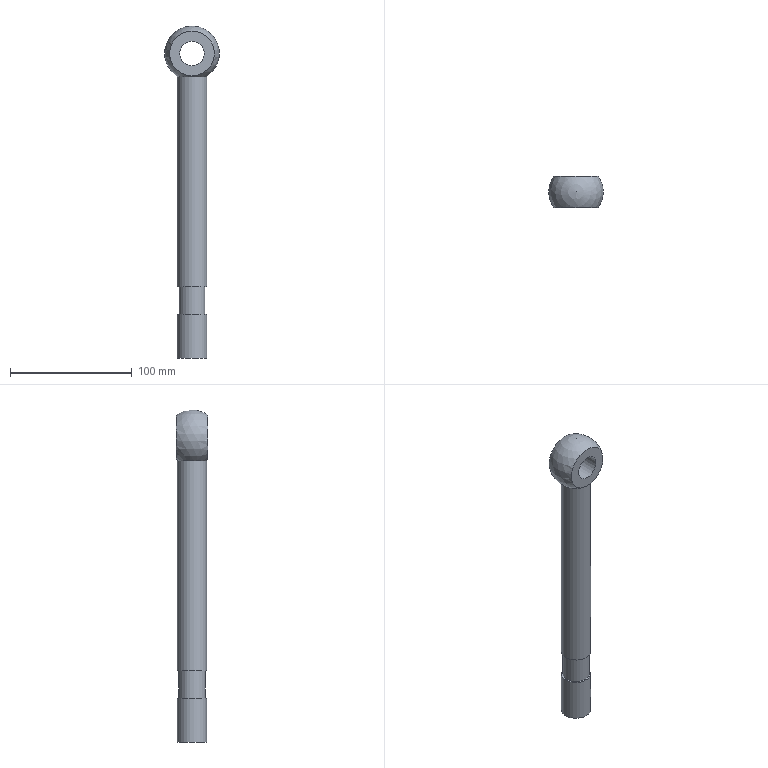Component | NX | HINGE_SCREW | 1 solid | 10 faces | box 45 x 26 x 272.5 mm | volume 130299 mm3 | plane 5 | cylinder 4 | sphere 1 | commonest cylinder face diameters 24 x2 20 x1 21.564 x1
STEP:
#1=CARTESIAN_POINT('',(0.,0.,0.));
#2=DIRECTION('',(0.,0.,1.));
#3=DIRECTION('',(1.,0.,0.));
#4=AXIS2_PLACEMENT_3D('',#1,#2,#3);
#5=CARTESIAN_POINT('',(-170.,-92.,248.467));
#6=VERTEX_POINT('',#5);
#7=CARTESIAN_POINT('',(-170.,-80.,248.467));
#8=DIRECTION('',(0.,0.,-1.));
#9=DIRECTION('',(0.,-1.,0.));
#10=AXIS2_PLACEMENT_3D('',#7,#8,#9);
#11=CIRCLE('',#10,12.);
#12=CARTESIAN_POINT('',(-170.,-80.,267.5));
#13=DIRECTION('',(0.,0.,1.));
#14=DIRECTION('',(0.,-1.,0.));
#15=AXIS2_PLACEMENT_3D('',#12,#13,#14);
#16=SPHERICAL_SURFACE('',#15,22.5);
#17=CARTESIAN_POINT('',(6.283,-1.008));
#18=CARTESIAN_POINT('',(6.188,-1.008));
#19=CARTESIAN_POINT('',(5.998,-1.008));
#20=CARTESIAN_POINT('',(5.712,-1.008));
#21=CARTESIAN_POINT('',(5.426,-1.008));
#22=CARTESIAN_POINT('',(5.141,-1.008));
#23=CARTESIAN_POINT('',(4.855,-1.008));
#24=CARTESIAN_POINT('',(4.57,-1.008));
#25=CARTESIAN_POINT('',(4.284,-1.008));
#26=CARTESIAN_POINT('',(3.998,-1.008));
#27=CARTESIAN_POINT('',(3.713,-1.008));
#28=CARTESIAN_POINT('',(3.427,-1.008));
#29=CARTESIAN_POINT('',(3.142,-1.008));
#30=CARTESIAN_POINT('',(2.856,-1.008));
#31=CARTESIAN_POINT('',(2.57,-1.008));
#32=CARTESIAN_POINT('',(2.285,-1.008));
#33=CARTESIAN_POINT('',(1.999,-1.008));
#34=CARTESIAN_POINT('',(1.714,-1.008));
#35=CARTESIAN_POINT('',(1.428,-1.008));
#36=CARTESIAN_POINT('',(1.142,-1.008));
#37=CARTESIAN_POINT('',(0.8568,-1.008));
#38=CARTESIAN_POINT('',(0.5712,-1.008));
#39=CARTESIAN_POINT('',(0.2856,-1.008));
#40=CARTESIAN_POINT('',(0.0952,-1.008));
#41=CARTESIAN_POINT('',(0.,-1.008));
#42=B_SPLINE_CURVE_WITH_KNOTS('',3,(#17,#18,#19,#20,#21,#22,#23,#24,#25,#26,#27,#28,#29,#30,#31,#32,#33,#34,#35,#36,#37,#38,#39,#40,#41),.UNSPECIFIED.,.F.,.F.,(4,1,1,1,1,1,1,1,1,1,1,1,1,1,1,1,1,1,1,1,1,1,4),(0.,0.2856,0.5712,0.8568,1.142,1.428,1.714,1.999,2.285,2.57,2.856,3.142,3.427,3.713,3.998,4.284,4.57,4.855,5.141,5.426,5.712,5.998,6.283),.QUASI_UNIFORM_KNOTS.);
#43=(GEOMETRIC_REPRESENTATION_CONTEXT(2)PARAMETRIC_REPRESENTATION_CONTEXT()REPRESENTATION_CONTEXT('',''));
#44=DEFINITIONAL_REPRESENTATION('',(#42),#43);
#45=PCURVE('',#16,#44);
#46=CARTESIAN_POINT('',(-170.,-80.,17.5));
#47=DIRECTION('',(0.,0.,1.));
#48=DIRECTION('',(0.,-1.,0.));
#49=AXIS2_PLACEMENT_3D('',#46,#47,#48);
#50=CYLINDRICAL_SURFACE('',#49,12.);
#51=CARTESIAN_POINT('',(6.283,230.967));
#52=DIRECTION('',(-1.,0.));
#53=VECTOR('',#52,1.);
#54=LINE('',#51,#53);
#55=(GEOMETRIC_REPRESENTATION_CONTEXT(2)PARAMETRIC_REPRESENTATION_CONTEXT()REPRESENTATION_CONTEXT('',''));
#56=DEFINITIONAL_REPRESENTATION('',(#54),#55);
#57=PCURVE('',#50,#56);
#58=SURFACE_CURVE('',#11,(#45,#57),.PCURVE_S1.);
#59=EDGE_CURVE('',#6,#6,#58,.T.);
#60=ORIENTED_EDGE('',*,*,#59,.F.);
#61=CARTESIAN_POINT('',(-170.,-93.,249.136));
#62=VERTEX_POINT('',#61);
#63=CARTESIAN_POINT('',(-170.,-92.,248.467));
#64=CARTESIAN_POINT('',(-170.,-92.339,248.681));
#65=CARTESIAN_POINT('',(-170.,-92.673,248.904));
#66=CARTESIAN_POINT('',(-170.,-93.,249.136));
#67=B_SPLINE_CURVE_WITH_KNOTS('',3,(#63,#64,#65,#66),.UNSPECIFIED.,.F.,.F.,(4,4),(-1.008,-0.9548),.PIECEWISE_BEZIER_KNOTS.);
#68=CARTESIAN_POINT('',(6.283,0.));
#69=DIRECTION('',(0.,1.));
#70=VECTOR('',#69,1.);
#71=LINE('',#68,#70);
#72=(GEOMETRIC_REPRESENTATION_CONTEXT(2)PARAMETRIC_REPRESENTATION_CONTEXT()REPRESENTATION_CONTEXT('',''));
#73=DEFINITIONAL_REPRESENTATION('',(#71),#72);
#74=PCURVE('',#16,#73);
#75=CARTESIAN_POINT('',(0.,0.));
#76=DIRECTION('',(0.,1.));
#77=VECTOR('',#76,1.);
#78=LINE('',#75,#77);
#79=(GEOMETRIC_REPRESENTATION_CONTEXT(2)PARAMETRIC_REPRESENTATION_CONTEXT()REPRESENTATION_CONTEXT('',''));
#80=DEFINITIONAL_REPRESENTATION('',(#78),#79);
#81=PCURVE('',#16,#80);
#82=SEAM_CURVE('',#67,(#74,#81),.PCURVE_S1.);
#83=EDGE_CURVE('',#6,#62,#82,.T.);
#84=ORIENTED_EDGE('',*,*,#83,.T.);
#85=CARTESIAN_POINT('',(-170.,-93.,285.864));
#86=VERTEX_POINT('',#85);
#87=CARTESIAN_POINT('',(-170.,-93.,267.5));
#88=DIRECTION('',(0.,1.,0.));
#89=DIRECTION('',(0.,0.,-1.));
#90=AXIS2_PLACEMENT_3D('',#87,#88,#89);
#91=CIRCLE('',#90,18.364);
#92=CARTESIAN_POINT('',(6.283,-0.9548));
#93=CARTESIAN_POINT('',(6.14,-0.9552));
#94=CARTESIAN_POINT('',(5.887,-0.9144));
#95=CARTESIAN_POINT('',(5.611,-0.7647));
#96=CARTESIAN_POINT('',(5.453,-0.5678));
#97=CARTESIAN_POINT('',(5.365,-0.3477));
#98=CARTESIAN_POINT('',(5.327,-0.1169));
#99=CARTESIAN_POINT('',(5.327,0.1169));
#100=CARTESIAN_POINT('',(5.366,0.3477));
#101=CARTESIAN_POINT('',(5.453,0.5678));
#102=CARTESIAN_POINT('',(5.612,0.7647));
#103=CARTESIAN_POINT('',(5.883,0.9147));
#104=CARTESIAN_POINT('',(6.283,0.9749));
#105=CARTESIAN_POINT('',(6.684,0.9147));
#106=CARTESIAN_POINT('',(6.954,0.7647));
#107=CARTESIAN_POINT('',(7.113,0.5678));
#108=CARTESIAN_POINT('',(7.201,0.3477));
#109=CARTESIAN_POINT('',(7.24,0.1169));
#110=CARTESIAN_POINT('',(7.24,-0.1169));
#111=CARTESIAN_POINT('',(7.201,-0.3477));
#112=CARTESIAN_POINT('',(7.113,-0.5678));
#113=CARTESIAN_POINT('',(6.955,-0.7647));
#114=CARTESIAN_POINT('',(6.679,-0.9144));
#115=CARTESIAN_POINT('',(6.427,-0.9552));
#116=CARTESIAN_POINT('',(6.283,-0.9548));
#117=B_SPLINE_CURVE_WITH_KNOTS('',3,(#92,#93,#94,#95,#96,#97,#98,#99,#100,#101,#102,#103,#104,#105,#106,#107,#108,#109,#110,#111,#112,#113,#114,#115,#116),.UNSPECIFIED.,.T.,.F.,(4,1,1,1,1,1,1,1,1,1,1,1,1,1,1,1,1,1,1,1,1,1,4),(0.,0.2856,0.5712,0.8568,1.142,1.428,1.714,1.999,2.285,2.57,2.856,3.142,3.427,3.713,3.998,4.284,4.57,4.855,5.141,5.426,5.712,5.998,6.283),.QUASI_UNIFORM_KNOTS.);
#118=(GEOMETRIC_REPRESENTATION_CONTEXT(2)PARAMETRIC_REPRESENTATION_CONTEXT()REPRESENTATION_CONTEXT('',''));
#119=DEFINITIONAL_REPRESENTATION('',(#117),#118);
#120=PCURVE('',#16,#119);
#121=CARTESIAN_POINT('',(-170.,-93.,267.5));
#122=DIRECTION('',(0.,-1.,0.));
#123=DIRECTION('',(0.,0.,-1.));
#124=AXIS2_PLACEMENT_3D('',#121,#122,#123);
#125=PLANE('',#124);
#126=CARTESIAN_POINT('',(18.364,0.));
#127=CARTESIAN_POINT('',(18.364,-31.808));
#128=CARTESIAN_POINT('',(-9.182,-15.904));
#129=CARTESIAN_POINT('',(-36.729,-0.));
#130=CARTESIAN_POINT('',(-9.182,15.904));
#131=CARTESIAN_POINT('',(18.364,31.808));
#132=CARTESIAN_POINT('',(18.364,0.));
#133=(BOUNDED_CURVE()B_SPLINE_CURVE(2,(#126,#127,#128,#129,#130,#131,#132),.UNSPECIFIED.,.T.,.F.)B_SPLINE_CURVE_WITH_KNOTS((1,2,2,2,2,1),(-2.094,0.,2.094,4.189,6.283,8.378),.UNSPECIFIED.)CURVE()GEOMETRIC_REPRESENTATION_ITEM()RATIONAL_B_SPLINE_CURVE((1.,0.5,1.,0.5,1.,0.5,1.))REPRESENTATION_ITEM(''));
#134=(GEOMETRIC_REPRESENTATION_CONTEXT(2)PARAMETRIC_REPRESENTATION_CONTEXT()REPRESENTATION_CONTEXT('',''));
#135=DEFINITIONAL_REPRESENTATION('',(#133),#134);
#136=PCURVE('',#125,#135);
#137=SURFACE_CURVE('',#91,(#120,#136),.PCURVE_S1.);
#138=EDGE_CURVE('',#62,#86,#137,.T.);
#139=ORIENTED_EDGE('',*,*,#138,.T.);
#140=CARTESIAN_POINT('',(-170.,-80.,290.));
#141=VERTEX_POINT('',#140);
#142=CARTESIAN_POINT('',(-170.,-93.,285.864));
#143=CARTESIAN_POINT('',(-170.,-90.737,287.466));
#144=CARTESIAN_POINT('',(-170.,-88.228,288.719));
#145=CARTESIAN_POINT('',(-170.,-85.544,289.573));
#146=CARTESIAN_POINT('',(-170.,-82.772,290.));
#147=CARTESIAN_POINT('',(-170.,-80.,290.));
#148=B_SPLINE_CURVE_WITH_KNOTS('',5,(#142,#143,#144,#145,#146,#147),.UNSPECIFIED.,.F.,.F.,(6,6),(0.9548,1.571),.PIECEWISE_BEZIER_KNOTS.);
#149=CARTESIAN_POINT('',(6.283,0.));
#150=DIRECTION('',(0.,1.));
#151=VECTOR('',#150,1.);
#152=LINE('',#149,#151);
#153=(GEOMETRIC_REPRESENTATION_CONTEXT(2)PARAMETRIC_REPRESENTATION_CONTEXT()REPRESENTATION_CONTEXT('',''));
#154=DEFINITIONAL_REPRESENTATION('',(#152),#153);
#155=PCURVE('',#16,#154);
#156=CARTESIAN_POINT('',(0.,0.));
#157=DIRECTION('',(0.,1.));
#158=VECTOR('',#157,1.);
#159=LINE('',#156,#158);
#160=(GEOMETRIC_REPRESENTATION_CONTEXT(2)PARAMETRIC_REPRESENTATION_CONTEXT()REPRESENTATION_CONTEXT('',''));
#161=DEFINITIONAL_REPRESENTATION('',(#159),#160);
#162=PCURVE('',#16,#161);
#163=SEAM_CURVE('',#148,(#155,#162),.PCURVE_S1.);
#164=EDGE_CURVE('',#86,#141,#163,.T.);
#165=ORIENTED_EDGE('',*,*,#164,.T.);
#166=ORIENTED_EDGE('',*,*,#164,.F.);
#167=CARTESIAN_POINT('',(-170.,-93.,267.5));
#168=DIRECTION('',(0.,1.,0.));
#169=DIRECTION('',(0.,0.,-1.));
#170=AXIS2_PLACEMENT_3D('',#167,#168,#169);
#171=CIRCLE('',#170,18.364);
#172=CARTESIAN_POINT('',(0.,-0.9548));
#173=CARTESIAN_POINT('',(-0.1436,-0.9552));
#174=CARTESIAN_POINT('',(-0.3958,-0.9144));
#175=CARTESIAN_POINT('',(-0.672,-0.7647));
#176=CARTESIAN_POINT('',(-0.8297,-0.5678));
#177=CARTESIAN_POINT('',(-0.9177,-0.3477));
#178=CARTESIAN_POINT('',(-0.9564,-0.1169));
#179=CARTESIAN_POINT('',(-0.9564,0.1169));
#180=CARTESIAN_POINT('',(-0.9176,0.3477));
#181=CARTESIAN_POINT('',(-0.83,0.5678));
#182=CARTESIAN_POINT('',(-0.6707,0.7647));
#183=CARTESIAN_POINT('',(-0.4005,0.9147));
#184=CARTESIAN_POINT('',(-0.,0.9749));
#185=CARTESIAN_POINT('',(0.4005,0.9147));
#186=CARTESIAN_POINT('',(0.6707,0.7647));
#187=CARTESIAN_POINT('',(0.83,0.5678));
#188=CARTESIAN_POINT('',(0.9176,0.3477));
#189=CARTESIAN_POINT('',(0.9564,0.1169));
#190=CARTESIAN_POINT('',(0.9564,-0.1169));
#191=CARTESIAN_POINT('',(0.9177,-0.3477));
#192=CARTESIAN_POINT('',(0.8297,-0.5678));
#193=CARTESIAN_POINT('',(0.672,-0.7647));
#194=CARTESIAN_POINT('',(0.3958,-0.9144));
#195=CARTESIAN_POINT('',(0.1436,-0.9552));
#196=CARTESIAN_POINT('',(0.,-0.9548));
#197=B_SPLINE_CURVE_WITH_KNOTS('',3,(#172,#173,#174,#175,#176,#177,#178,#179,#180,#181,#182,#183,#184,#185,#186,#187,#188,#189,#190,#191,#192,#193,#194,#195,#196),.UNSPECIFIED.,.T.,.F.,(4,1,1,1,1,1,1,1,1,1,1,1,1,1,1,1,1,1,1,1,1,1,4),(0.,0.2856,0.5712,0.8568,1.142,1.428,1.714,1.999,2.285,2.57,2.856,3.142,3.427,3.713,3.998,4.284,4.57,4.855,5.141,5.426,5.712,5.998,6.283),.QUASI_UNIFORM_KNOTS.);
#198=(GEOMETRIC_REPRESENTATION_CONTEXT(2)PARAMETRIC_REPRESENTATION_CONTEXT()REPRESENTATION_CONTEXT('',''));
#199=DEFINITIONAL_REPRESENTATION('',(#197),#198);
#200=PCURVE('',#16,#199);
#201=CARTESIAN_POINT('',(18.364,0.));
#202=CARTESIAN_POINT('',(18.364,-31.808));
#203=CARTESIAN_POINT('',(-9.182,-15.904));
#204=CARTESIAN_POINT('',(-36.729,-0.));
#205=CARTESIAN_POINT('',(-9.182,15.904));
#206=CARTESIAN_POINT('',(18.364,31.808));
#207=CARTESIAN_POINT('',(18.364,0.));
#208=(BOUNDED_CURVE()B_SPLINE_CURVE(2,(#201,#202,#203,#204,#205,#206,#207),.UNSPECIFIED.,.T.,.F.)B_SPLINE_CURVE_WITH_KNOTS((1,2,2,2,2,1),(-2.094,0.,2.094,4.189,6.283,8.378),.UNSPECIFIED.)CURVE()GEOMETRIC_REPRESENTATION_ITEM()RATIONAL_B_SPLINE_CURVE((1.,0.5,1.,0.5,1.,0.5,1.))REPRESENTATION_ITEM(''));
#209=(GEOMETRIC_REPRESENTATION_CONTEXT(2)PARAMETRIC_REPRESENTATION_CONTEXT()REPRESENTATION_CONTEXT('',''));
#210=DEFINITIONAL_REPRESENTATION('',(#208),#209);
#211=PCURVE('',#125,#210);
#212=SURFACE_CURVE('',#171,(#200,#211),.PCURVE_S1.);
#213=EDGE_CURVE('',#86,#62,#212,.T.);
#214=ORIENTED_EDGE('',*,*,#213,.T.);
#215=ORIENTED_EDGE('',*,*,#83,.F.);
#216=EDGE_LOOP('',(#60,#84,#139,#165,#166,#214,#215));
#217=FACE_BOUND('',#216,.T.);
#218=CARTESIAN_POINT('',(-170.,-67.,285.864));
#219=VERTEX_POINT('',#218);
#220=CARTESIAN_POINT('',(-170.,-67.,267.5));
#221=DIRECTION('',(0.,-1.,0.));
#222=DIRECTION('',(0.,0.,1.));
#223=AXIS2_PLACEMENT_3D('',#220,#221,#222);
#224=CIRCLE('',#223,18.364);
#225=CARTESIAN_POINT('',(3.142,0.9548));
#226=CARTESIAN_POINT('',(3.285,0.9552));
#227=CARTESIAN_POINT('',(3.537,0.9144));
#228=CARTESIAN_POINT('',(3.814,0.7647));
#229=CARTESIAN_POINT('',(3.971,0.5678));
#230=CARTESIAN_POINT('',(4.059,0.3477));
#231=CARTESIAN_POINT('',(4.098,0.1169));
#232=CARTESIAN_POINT('',(4.098,-0.1169));
#233=CARTESIAN_POINT('',(4.059,-0.3477));
#234=CARTESIAN_POINT('',(3.972,-0.5678));
#235=CARTESIAN_POINT('',(3.812,-0.7647));
#236=CARTESIAN_POINT('',(3.542,-0.9147));
#237=CARTESIAN_POINT('',(3.142,-0.9749));
#238=CARTESIAN_POINT('',(2.741,-0.9147));
#239=CARTESIAN_POINT('',(2.471,-0.7647));
#240=CARTESIAN_POINT('',(2.312,-0.5678));
#241=CARTESIAN_POINT('',(2.224,-0.3477));
#242=CARTESIAN_POINT('',(2.185,-0.1169));
#243=CARTESIAN_POINT('',(2.185,0.1169));
#244=CARTESIAN_POINT('',(2.224,0.3477));
#245=CARTESIAN_POINT('',(2.312,0.5678));
#246=CARTESIAN_POINT('',(2.47,0.7647));
#247=CARTESIAN_POINT('',(2.746,0.9144));
#248=CARTESIAN_POINT('',(2.998,0.9552));
#249=CARTESIAN_POINT('',(3.142,0.9548));
#250=B_SPLINE_CURVE_WITH_KNOTS('',3,(#225,#226,#227,#228,#229,#230,#231,#232,#233,#234,#235,#236,#237,#238,#239,#240,#241,#242,#243,#244,#245,#246,#247,#248,#249),.UNSPECIFIED.,.T.,.F.,(4,1,1,1,1,1,1,1,1,1,1,1,1,1,1,1,1,1,1,1,1,1,4),(0.,0.2856,0.5712,0.8568,1.142,1.428,1.714,1.999,2.285,2.57,2.856,3.142,3.427,3.713,3.998,4.284,4.57,4.855,5.141,5.426,5.712,5.998,6.283),.QUASI_UNIFORM_KNOTS.);
#251=(GEOMETRIC_REPRESENTATION_CONTEXT(2)PARAMETRIC_REPRESENTATION_CONTEXT()REPRESENTATION_CONTEXT('',''));
#252=DEFINITIONAL_REPRESENTATION('',(#250),#251);
#253=PCURVE('',#16,#252);
#254=CARTESIAN_POINT('',(-170.,-67.,267.5));
#255=DIRECTION('',(0.,1.,0.));
#256=DIRECTION('',(0.,0.,1.));
#257=AXIS2_PLACEMENT_3D('',#254,#255,#256);
#258=PLANE('',#257);
#259=CARTESIAN_POINT('',(18.364,0.));
#260=CARTESIAN_POINT('',(18.364,-31.808));
#261=CARTESIAN_POINT('',(-9.182,-15.904));
#262=CARTESIAN_POINT('',(-36.729,-0.));
#263=CARTESIAN_POINT('',(-9.182,15.904));
#264=CARTESIAN_POINT('',(18.364,31.808));
#265=CARTESIAN_POINT('',(18.364,0.));
#266=(BOUNDED_CURVE()B_SPLINE_CURVE(2,(#259,#260,#261,#262,#263,#264,#265),.UNSPECIFIED.,.T.,.F.)B_SPLINE_CURVE_WITH_KNOTS((1,2,2,2,2,1),(-2.094,0.,2.094,4.189,6.283,8.378),.UNSPECIFIED.)CURVE()GEOMETRIC_REPRESENTATION_ITEM()RATIONAL_B_SPLINE_CURVE((1.,0.5,1.,0.5,1.,0.5,1.))REPRESENTATION_ITEM(''));
#267=(GEOMETRIC_REPRESENTATION_CONTEXT(2)PARAMETRIC_REPRESENTATION_CONTEXT()REPRESENTATION_CONTEXT('',''));
#268=DEFINITIONAL_REPRESENTATION('',(#266),#267);
#269=PCURVE('',#258,#268);
#270=SURFACE_CURVE('',#224,(#253,#269),.PCURVE_S1.);
#271=EDGE_CURVE('',#219,#219,#270,.T.);
#272=ORIENTED_EDGE('',*,*,#271,.T.);
#273=EDGE_LOOP('',(#272));
#274=FACE_BOUND('',#273,.T.);
#275=ADVANCED_FACE('',(#217,#274),#16,.T.);
#276=CARTESIAN_POINT('',(-170.,-93.,277.5));
#277=VERTEX_POINT('',#276);
#278=CARTESIAN_POINT('',(-170.,-93.,267.5));
#279=DIRECTION('',(0.,1.,0.));
#280=DIRECTION('',(0.,0.,1.));
#281=AXIS2_PLACEMENT_3D('',#278,#279,#280);
#282=CIRCLE('',#281,10.);
#283=CARTESIAN_POINT('',(-10.,0.));
#284=CARTESIAN_POINT('',(-10.,17.321));
#285=CARTESIAN_POINT('',(5.,8.66));
#286=CARTESIAN_POINT('',(20.,0.));
#287=CARTESIAN_POINT('',(5.,-8.66));
#288=CARTESIAN_POINT('',(-10.,-17.321));
#289=CARTESIAN_POINT('',(-10.,0.));
#290=(BOUNDED_CURVE()B_SPLINE_CURVE(2,(#283,#284,#285,#286,#287,#288,#289),.UNSPECIFIED.,.T.,.F.)B_SPLINE_CURVE_WITH_KNOTS((1,2,2,2,2,1),(-2.094,0.,2.094,4.189,6.283,8.378),.UNSPECIFIED.)CURVE()GEOMETRIC_REPRESENTATION_ITEM()RATIONAL_B_SPLINE_CURVE((1.,0.5,1.,0.5,1.,0.5,1.))REPRESENTATION_ITEM(''));
#291=(GEOMETRIC_REPRESENTATION_CONTEXT(2)PARAMETRIC_REPRESENTATION_CONTEXT()REPRESENTATION_CONTEXT('',''));
#292=DEFINITIONAL_REPRESENTATION('',(#290),#291);
#293=PCURVE('',#125,#292);
#294=CARTESIAN_POINT('',(-170.,-93.,267.5));
#295=DIRECTION('',(0.,1.,0.));
#296=DIRECTION('',(0.,0.,1.));
#297=AXIS2_PLACEMENT_3D('',#294,#295,#296);
#298=CYLINDRICAL_SURFACE('',#297,10.);
#299=CARTESIAN_POINT('',(0.,0.));
#300=DIRECTION('',(1.,0.));
#301=VECTOR('',#300,1.);
#302=LINE('',#299,#301);
#303=(GEOMETRIC_REPRESENTATION_CONTEXT(2)PARAMETRIC_REPRESENTATION_CONTEXT()REPRESENTATION_CONTEXT('',''));
#304=DEFINITIONAL_REPRESENTATION('',(#302),#303);
#305=PCURVE('',#298,#304);
#306=SURFACE_CURVE('',#282,(#293,#305),.PCURVE_S1.);
#307=EDGE_CURVE('',#277,#277,#306,.T.);
#308=ORIENTED_EDGE('',*,*,#307,.T.);
#309=EDGE_LOOP('',(#308));
#310=FACE_BOUND('',#309,.T.);
#311=ORIENTED_EDGE('',*,*,#138,.F.);
#312=ORIENTED_EDGE('',*,*,#213,.F.);
#313=EDGE_LOOP('',(#311,#312));
#314=FACE_BOUND('',#313,.T.);
#315=ADVANCED_FACE('',(#310,#314),#125,.T.);
#316=CARTESIAN_POINT('',(-170.,-67.,277.5));
#317=VERTEX_POINT('',#316);
#318=CARTESIAN_POINT('',(-170.,-67.,267.5));
#319=DIRECTION('',(0.,1.,0.));
#320=DIRECTION('',(0.,0.,1.));
#321=AXIS2_PLACEMENT_3D('',#318,#319,#320);
#322=CIRCLE('',#321,10.);
#323=CARTESIAN_POINT('',(0.,0.));
#324=DIRECTION('',(1.,0.));
#325=AXIS2_PLACEMENT_2D('',#323,#324);
#326=CIRCLE('',#325,10.);
#327=(GEOMETRIC_REPRESENTATION_CONTEXT(2)PARAMETRIC_REPRESENTATION_CONTEXT()REPRESENTATION_CONTEXT('',''));
#328=DEFINITIONAL_REPRESENTATION('',(#326),#327);
#329=PCURVE('',#258,#328);
#330=CARTESIAN_POINT('',(0.,26.));
#331=DIRECTION('',(1.,0.));
#332=VECTOR('',#331,1.);
#333=LINE('',#330,#332);
#334=(GEOMETRIC_REPRESENTATION_CONTEXT(2)PARAMETRIC_REPRESENTATION_CONTEXT()REPRESENTATION_CONTEXT('',''));
#335=DEFINITIONAL_REPRESENTATION('',(#333),#334);
#336=PCURVE('',#298,#335);
#337=SURFACE_CURVE('',#322,(#329,#336),.PCURVE_S1.);
#338=EDGE_CURVE('',#317,#317,#337,.T.);
#339=ORIENTED_EDGE('',*,*,#338,.F.);
#340=EDGE_LOOP('',(#339));
#341=FACE_BOUND('',#340,.T.);
#342=ORIENTED_EDGE('',*,*,#271,.F.);
#343=EDGE_LOOP('',(#342));
#344=FACE_BOUND('',#343,.T.);
#345=ADVANCED_FACE('',(#341,#344),#258,.T.);
#346=CARTESIAN_POINT('',(-170.,-92.,76.));
#347=VERTEX_POINT('',#346);
#348=CARTESIAN_POINT('',(-170.,-80.,76.));
#349=DIRECTION('',(0.,0.,-1.));
#350=DIRECTION('',(0.,-1.,0.));
#351=AXIS2_PLACEMENT_3D('',#348,#349,#350);
#352=CIRCLE('',#351,12.);
#353=CARTESIAN_POINT('',(6.283,58.5));
#354=DIRECTION('',(-1.,0.));
#355=VECTOR('',#354,1.);
#356=LINE('',#353,#355);
#357=(GEOMETRIC_REPRESENTATION_CONTEXT(2)PARAMETRIC_REPRESENTATION_CONTEXT()REPRESENTATION_CONTEXT('',''));
#358=DEFINITIONAL_REPRESENTATION('',(#356),#357);
#359=PCURVE('',#50,#358);
#360=CARTESIAN_POINT('',(-170.,-80.,76.));
#361=DIRECTION('',(0.,0.,1.));
#362=DIRECTION('',(0.,-1.,0.));
#363=AXIS2_PLACEMENT_3D('',#360,#361,#362);
#364=PLANE('',#363);
#365=CARTESIAN_POINT('',(12.,0.));
#366=CARTESIAN_POINT('',(12.,-20.785));
#367=CARTESIAN_POINT('',(-6.,-10.392));
#368=CARTESIAN_POINT('',(-24.,-0.));
#369=CARTESIAN_POINT('',(-6.,10.392));
#370=CARTESIAN_POINT('',(12.,20.785));
#371=CARTESIAN_POINT('',(12.,0.));
#372=(BOUNDED_CURVE()B_SPLINE_CURVE(2,(#365,#366,#367,#368,#369,#370,#371),.UNSPECIFIED.,.T.,.F.)B_SPLINE_CURVE_WITH_KNOTS((1,2,2,2,2,1),(-2.094,0.,2.094,4.189,6.283,8.378),.UNSPECIFIED.)CURVE()GEOMETRIC_REPRESENTATION_ITEM()RATIONAL_B_SPLINE_CURVE((1.,0.5,1.,0.5,1.,0.5,1.))REPRESENTATION_ITEM(''));
#373=(GEOMETRIC_REPRESENTATION_CONTEXT(2)PARAMETRIC_REPRESENTATION_CONTEXT()REPRESENTATION_CONTEXT('',''));
#374=DEFINITIONAL_REPRESENTATION('',(#372),#373);
#375=PCURVE('',#364,#374);
#376=SURFACE_CURVE('',#352,(#359,#375),.PCURVE_S1.);
#377=EDGE_CURVE('',#347,#347,#376,.T.);
#378=ORIENTED_EDGE('',*,*,#377,.F.);
#379=CARTESIAN_POINT('',(-170.,-92.,76.));
#380=CARTESIAN_POINT('',(-170.,-92.,248.467));
#381=B_SPLINE_CURVE_WITH_KNOTS('',1,(#379,#380),.UNSPECIFIED.,.F.,.F.,(2,2),(58.5,230.967),.PIECEWISE_BEZIER_KNOTS.);
#382=CARTESIAN_POINT('',(6.283,0.));
#383=DIRECTION('',(0.,1.));
#384=VECTOR('',#383,1.);
#385=LINE('',#382,#384);
#386=(GEOMETRIC_REPRESENTATION_CONTEXT(2)PARAMETRIC_REPRESENTATION_CONTEXT()REPRESENTATION_CONTEXT('',''));
#387=DEFINITIONAL_REPRESENTATION('',(#385),#386);
#388=PCURVE('',#50,#387);
#389=CARTESIAN_POINT('',(0.,0.));
#390=DIRECTION('',(0.,1.));
#391=VECTOR('',#390,1.);
#392=LINE('',#389,#391);
#393=(GEOMETRIC_REPRESENTATION_CONTEXT(2)PARAMETRIC_REPRESENTATION_CONTEXT()REPRESENTATION_CONTEXT('',''));
#394=DEFINITIONAL_REPRESENTATION('',(#392),#393);
#395=PCURVE('',#50,#394);
#396=SEAM_CURVE('',#381,(#388,#395),.PCURVE_S1.);
#397=EDGE_CURVE('',#347,#6,#396,.T.);
#398=ORIENTED_EDGE('',*,*,#397,.T.);
#399=ORIENTED_EDGE('',*,*,#59,.T.);
#400=ORIENTED_EDGE('',*,*,#397,.F.);
#401=EDGE_LOOP('',(#378,#398,#399,#400));
#402=FACE_BOUND('',#401,.T.);
#403=ADVANCED_FACE('',(#402),#50,.T.);
#404=ORIENTED_EDGE('',*,*,#338,.F.);
#405=CARTESIAN_POINT('',(-170.,-93.,277.5));
#406=CARTESIAN_POINT('',(-170.,-67.,277.5));
#407=B_SPLINE_CURVE_WITH_KNOTS('',1,(#405,#406),.UNSPECIFIED.,.F.,.F.,(2,2),(0.,26.),.PIECEWISE_BEZIER_KNOTS.);
#408=CARTESIAN_POINT('',(0.,0.));
#409=DIRECTION('',(0.,1.));
#410=VECTOR('',#409,1.);
#411=LINE('',#408,#410);
#412=(GEOMETRIC_REPRESENTATION_CONTEXT(2)PARAMETRIC_REPRESENTATION_CONTEXT()REPRESENTATION_CONTEXT('',''));
#413=DEFINITIONAL_REPRESENTATION('',(#411),#412);
#414=PCURVE('',#298,#413);
#415=CARTESIAN_POINT('',(6.283,0.));
#416=DIRECTION('',(0.,1.));
#417=VECTOR('',#416,1.);
#418=LINE('',#415,#417);
#419=(GEOMETRIC_REPRESENTATION_CONTEXT(2)PARAMETRIC_REPRESENTATION_CONTEXT()REPRESENTATION_CONTEXT('',''));
#420=DEFINITIONAL_REPRESENTATION('',(#418),#419);
#421=PCURVE('',#298,#420);
#422=SEAM_CURVE('',#407,(#414,#421),.PCURVE_S1.);
#423=EDGE_CURVE('',#277,#317,#422,.T.);
#424=ORIENTED_EDGE('',*,*,#423,.F.);
#425=ORIENTED_EDGE('',*,*,#307,.T.);
#426=ORIENTED_EDGE('',*,*,#423,.T.);
#427=EDGE_LOOP('',(#404,#424,#425,#426));
#428=FACE_BOUND('',#427,.F.);
#429=ADVANCED_FACE('',(#428),#298,.F.);
#430=CARTESIAN_POINT('',(-170.,-90.782,76.));
#431=VERTEX_POINT('',#430);
#432=CARTESIAN_POINT('',(-170.,-80.,76.));
#433=DIRECTION('',(0.,0.,1.));
#434=DIRECTION('',(0.,-1.,0.));
#435=AXIS2_PLACEMENT_3D('',#432,#433,#434);
#436=CIRCLE('',#435,10.782);
#437=CARTESIAN_POINT('',(-170.,-80.,76.));
#438=DIRECTION('',(0.,0.,-1.));
#439=DIRECTION('',(0.,1.,0.));
#440=AXIS2_PLACEMENT_3D('',#437,#438,#439);
#441=CYLINDRICAL_SURFACE('',#440,10.782);
#442=CARTESIAN_POINT('',(9.425,0.));
#443=DIRECTION('',(-1.,0.));
#444=VECTOR('',#443,1.);
#445=LINE('',#442,#444);
#446=(GEOMETRIC_REPRESENTATION_CONTEXT(2)PARAMETRIC_REPRESENTATION_CONTEXT()REPRESENTATION_CONTEXT('',''));
#447=DEFINITIONAL_REPRESENTATION('',(#445),#446);
#448=PCURVE('',#441,#447);
#449=CARTESIAN_POINT('',(0.,0.));
#450=DIRECTION('',(1.,0.));
#451=AXIS2_PLACEMENT_2D('',#449,#450);
#452=CIRCLE('',#451,10.782);
#453=(GEOMETRIC_REPRESENTATION_CONTEXT(2)PARAMETRIC_REPRESENTATION_CONTEXT()REPRESENTATION_CONTEXT('',''));
#454=DEFINITIONAL_REPRESENTATION('',(#452),#453);
#455=PCURVE('',#364,#454);
#456=SURFACE_CURVE('',#436,(#448,#455),.PCURVE_S1.);
#457=EDGE_CURVE('',#431,#431,#456,.T.);
#458=ORIENTED_EDGE('',*,*,#457,.F.);
#459=CARTESIAN_POINT('',(-170.,-90.782,53.5));
#460=VERTEX_POINT('',#459);
#461=CARTESIAN_POINT('',(-170.,-90.782,76.));
#462=CARTESIAN_POINT('',(-170.,-90.782,53.5));
#463=B_SPLINE_CURVE_WITH_KNOTS('',1,(#461,#462),.UNSPECIFIED.,.F.,.F.,(2,2),(0.,22.5),.PIECEWISE_BEZIER_KNOTS.);
#464=CARTESIAN_POINT('',(9.425,0.));
#465=DIRECTION('',(0.,1.));
#466=VECTOR('',#465,1.);
#467=LINE('',#464,#466);
#468=(GEOMETRIC_REPRESENTATION_CONTEXT(2)PARAMETRIC_REPRESENTATION_CONTEXT()REPRESENTATION_CONTEXT('',''));
#469=DEFINITIONAL_REPRESENTATION('',(#467),#468);
#470=PCURVE('',#441,#469);
#471=CARTESIAN_POINT('',(3.142,0.));
#472=DIRECTION('',(0.,1.));
#473=VECTOR('',#472,1.);
#474=LINE('',#471,#473);
#475=(GEOMETRIC_REPRESENTATION_CONTEXT(2)PARAMETRIC_REPRESENTATION_CONTEXT()REPRESENTATION_CONTEXT('',''));
#476=DEFINITIONAL_REPRESENTATION('',(#474),#475);
#477=PCURVE('',#441,#476);
#478=SEAM_CURVE('',#463,(#470,#477),.PCURVE_S1.);
#479=EDGE_CURVE('',#431,#460,#478,.T.);
#480=ORIENTED_EDGE('',*,*,#479,.T.);
#481=CARTESIAN_POINT('',(-170.,-80.,53.5));
#482=DIRECTION('',(0.,0.,1.));
#483=DIRECTION('',(0.,-1.,0.));
#484=AXIS2_PLACEMENT_3D('',#481,#482,#483);
#485=CIRCLE('',#484,10.782);
#486=CARTESIAN_POINT('',(9.425,22.5));
#487=DIRECTION('',(-1.,0.));
#488=VECTOR('',#487,1.);
#489=LINE('',#486,#488);
#490=(GEOMETRIC_REPRESENTATION_CONTEXT(2)PARAMETRIC_REPRESENTATION_CONTEXT()REPRESENTATION_CONTEXT('',''));
#491=DEFINITIONAL_REPRESENTATION('',(#489),#490);
#492=PCURVE('',#441,#491);
#493=CARTESIAN_POINT('',(-170.,-80.,53.5));
#494=DIRECTION('',(0.,0.,1.));
#495=DIRECTION('',(0.,-1.,0.));
#496=AXIS2_PLACEMENT_3D('',#493,#494,#495);
#497=PLANE('',#496);
#498=CARTESIAN_POINT('',(0.,0.));
#499=DIRECTION('',(1.,0.));
#500=AXIS2_PLACEMENT_2D('',#498,#499);
#501=CIRCLE('',#500,10.782);
#502=(GEOMETRIC_REPRESENTATION_CONTEXT(2)PARAMETRIC_REPRESENTATION_CONTEXT()REPRESENTATION_CONTEXT('',''));
#503=DEFINITIONAL_REPRESENTATION('',(#501),#502);
#504=PCURVE('',#497,#503);
#505=SURFACE_CURVE('',#485,(#492,#504),.PCURVE_S1.);
#506=EDGE_CURVE('',#460,#460,#505,.T.);
#507=ORIENTED_EDGE('',*,*,#506,.T.);
#508=ORIENTED_EDGE('',*,*,#479,.F.);
#509=EDGE_LOOP('',(#458,#480,#507,#508));
#510=FACE_BOUND('',#509,.T.);
#511=ADVANCED_FACE('',(#510),#441,.T.);
#512=ORIENTED_EDGE('',*,*,#377,.T.);
#513=EDGE_LOOP('',(#512));
#514=FACE_BOUND('',#513,.T.);
#515=ORIENTED_EDGE('',*,*,#457,.T.);
#516=EDGE_LOOP('',(#515));
#517=FACE_BOUND('',#516,.T.);
#518=ADVANCED_FACE('',(#514,#517),#364,.F.);
#519=CARTESIAN_POINT('',(-170.,-92.,53.5));
#520=VERTEX_POINT('',#519);
#521=CARTESIAN_POINT('',(-170.,-80.,53.5));
#522=DIRECTION('',(0.,0.,-1.));
#523=DIRECTION('',(0.,-1.,0.));
#524=AXIS2_PLACEMENT_3D('',#521,#522,#523);
#525=CIRCLE('',#524,12.);
#526=CARTESIAN_POINT('',(12.,0.));
#527=CARTESIAN_POINT('',(12.,-20.785));
#528=CARTESIAN_POINT('',(-6.,-10.392));
#529=CARTESIAN_POINT('',(-24.,-0.));
#530=CARTESIAN_POINT('',(-6.,10.392));
#531=CARTESIAN_POINT('',(12.,20.785));
#532=CARTESIAN_POINT('',(12.,0.));
#533=(BOUNDED_CURVE()B_SPLINE_CURVE(2,(#526,#527,#528,#529,#530,#531,#532),.UNSPECIFIED.,.T.,.F.)B_SPLINE_CURVE_WITH_KNOTS((1,2,2,2,2,1),(-2.094,0.,2.094,4.189,6.283,8.378),.UNSPECIFIED.)CURVE()GEOMETRIC_REPRESENTATION_ITEM()RATIONAL_B_SPLINE_CURVE((1.,0.5,1.,0.5,1.,0.5,1.))REPRESENTATION_ITEM(''));
#534=(GEOMETRIC_REPRESENTATION_CONTEXT(2)PARAMETRIC_REPRESENTATION_CONTEXT()REPRESENTATION_CONTEXT('',''));
#535=DEFINITIONAL_REPRESENTATION('',(#533),#534);
#536=PCURVE('',#497,#535);
#537=CARTESIAN_POINT('',(-170.,-80.,17.5));
#538=DIRECTION('',(0.,0.,1.));
#539=DIRECTION('',(0.,-1.,0.));
#540=AXIS2_PLACEMENT_3D('',#537,#538,#539);
#541=CYLINDRICAL_SURFACE('',#540,12.);
#542=CARTESIAN_POINT('',(6.283,36.));
#543=DIRECTION('',(-1.,0.));
#544=VECTOR('',#543,1.);
#545=LINE('',#542,#544);
#546=(GEOMETRIC_REPRESENTATION_CONTEXT(2)PARAMETRIC_REPRESENTATION_CONTEXT()REPRESENTATION_CONTEXT('',''));
#547=DEFINITIONAL_REPRESENTATION('',(#545),#546);
#548=PCURVE('',#541,#547);
#549=SURFACE_CURVE('',#525,(#536,#548),.PCURVE_S1.);
#550=EDGE_CURVE('',#520,#520,#549,.T.);
#551=ORIENTED_EDGE('',*,*,#550,.F.);
#552=EDGE_LOOP('',(#551));
#553=FACE_BOUND('',#552,.T.);
#554=ORIENTED_EDGE('',*,*,#506,.F.);
#555=EDGE_LOOP('',(#554));
#556=FACE_BOUND('',#555,.T.);
#557=ADVANCED_FACE('',(#553,#556),#497,.T.);
#558=CARTESIAN_POINT('',(-170.,-92.,17.5));
#559=VERTEX_POINT('',#558);
#560=CARTESIAN_POINT('',(-170.,-80.,17.5));
#561=DIRECTION('',(0.,0.,1.));
#562=DIRECTION('',(0.,-1.,0.));
#563=AXIS2_PLACEMENT_3D('',#560,#561,#562);
#564=CIRCLE('',#563,12.);
#565=CARTESIAN_POINT('',(-170.,-80.,17.5));
#566=DIRECTION('',(0.,0.,1.));
#567=DIRECTION('',(0.,-1.,0.));
#568=AXIS2_PLACEMENT_3D('',#565,#566,#567);
#569=PLANE('',#568);
#570=CARTESIAN_POINT('',(0.,0.));
#571=DIRECTION('',(1.,0.));
#572=AXIS2_PLACEMENT_2D('',#570,#571);
#573=CIRCLE('',#572,12.);
#574=(GEOMETRIC_REPRESENTATION_CONTEXT(2)PARAMETRIC_REPRESENTATION_CONTEXT()REPRESENTATION_CONTEXT('',''));
#575=DEFINITIONAL_REPRESENTATION('',(#573),#574);
#576=PCURVE('',#569,#575);
#577=CARTESIAN_POINT('',(0.,0.));
#578=DIRECTION('',(1.,0.));
#579=VECTOR('',#578,1.);
#580=LINE('',#577,#579);
#581=(GEOMETRIC_REPRESENTATION_CONTEXT(2)PARAMETRIC_REPRESENTATION_CONTEXT()REPRESENTATION_CONTEXT('',''));
#582=DEFINITIONAL_REPRESENTATION('',(#580),#581);
#583=PCURVE('',#541,#582);
#584=SURFACE_CURVE('',#564,(#576,#583),.PCURVE_S1.);
#585=EDGE_CURVE('',#559,#559,#584,.T.);
#586=ORIENTED_EDGE('',*,*,#585,.F.);
#587=EDGE_LOOP('',(#586));
#588=FACE_BOUND('',#587,.T.);
#589=ADVANCED_FACE('',(#588),#569,.F.);
#590=ORIENTED_EDGE('',*,*,#585,.T.);
#591=CARTESIAN_POINT('',(-170.,-92.,17.5));
#592=CARTESIAN_POINT('',(-170.,-92.,53.5));
#593=B_SPLINE_CURVE_WITH_KNOTS('',1,(#591,#592),.UNSPECIFIED.,.F.,.F.,(2,2),(0.,36.),.PIECEWISE_BEZIER_KNOTS.);
#594=CARTESIAN_POINT('',(6.283,0.));
#595=DIRECTION('',(0.,1.));
#596=VECTOR('',#595,1.);
#597=LINE('',#594,#596);
#598=(GEOMETRIC_REPRESENTATION_CONTEXT(2)PARAMETRIC_REPRESENTATION_CONTEXT()REPRESENTATION_CONTEXT('',''));
#599=DEFINITIONAL_REPRESENTATION('',(#597),#598);
#600=PCURVE('',#541,#599);
#601=CARTESIAN_POINT('',(0.,0.));
#602=DIRECTION('',(0.,1.));
#603=VECTOR('',#602,1.);
#604=LINE('',#601,#603);
#605=(GEOMETRIC_REPRESENTATION_CONTEXT(2)PARAMETRIC_REPRESENTATION_CONTEXT()REPRESENTATION_CONTEXT('',''));
#606=DEFINITIONAL_REPRESENTATION('',(#604),#605);
#607=PCURVE('',#541,#606);
#608=SEAM_CURVE('',#593,(#600,#607),.PCURVE_S1.);
#609=EDGE_CURVE('',#559,#520,#608,.T.);
#610=ORIENTED_EDGE('',*,*,#609,.T.);
#611=ORIENTED_EDGE('',*,*,#550,.T.);
#612=ORIENTED_EDGE('',*,*,#609,.F.);
#613=EDGE_LOOP('',(#590,#610,#611,#612));
#614=FACE_BOUND('',#613,.T.);
#615=ADVANCED_FACE('',(#614),#541,.T.);
#616=CLOSED_SHELL('',(#275,#315,#345,#403,#429,#511,#518,#557,#589,#615));
#617=MANIFOLD_SOLID_BREP('',#616);
#618=(LENGTH_UNIT()NAMED_UNIT(*)SI_UNIT(.MILLI.,.METRE.));
#619=UNCERTAINTY_MEASURE_WITH_UNIT(LENGTH_MEASURE(0.01),#618,'','');
#620=(NAMED_UNIT(*)PLANE_ANGLE_UNIT()SI_UNIT($,.RADIAN.));
#621=(NAMED_UNIT(*)SI_UNIT($,.STERADIAN.)SOLID_ANGLE_UNIT());
#622=(GEOMETRIC_REPRESENTATION_CONTEXT(3)GLOBAL_UNCERTAINTY_ASSIGNED_CONTEXT((#619))GLOBAL_UNIT_ASSIGNED_CONTEXT((#618,#620,#621))REPRESENTATION_CONTEXT('',''));
#623=ADVANCED_BREP_SHAPE_REPRESENTATION('',(#4,#617),#622);